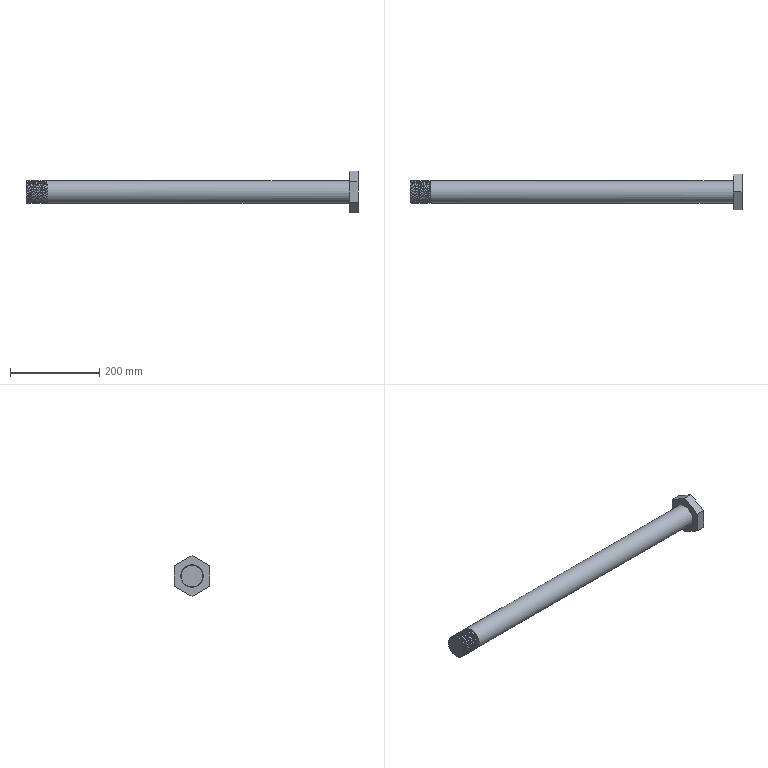Component | NX | PIN_SHAFT_2_2 | 1 solid | 24 faces | volume 1532057 mm3 | cylinder 12 | plane 10 | spline 2 | commonest cylinder face diameters 50 x11 48.5 x1